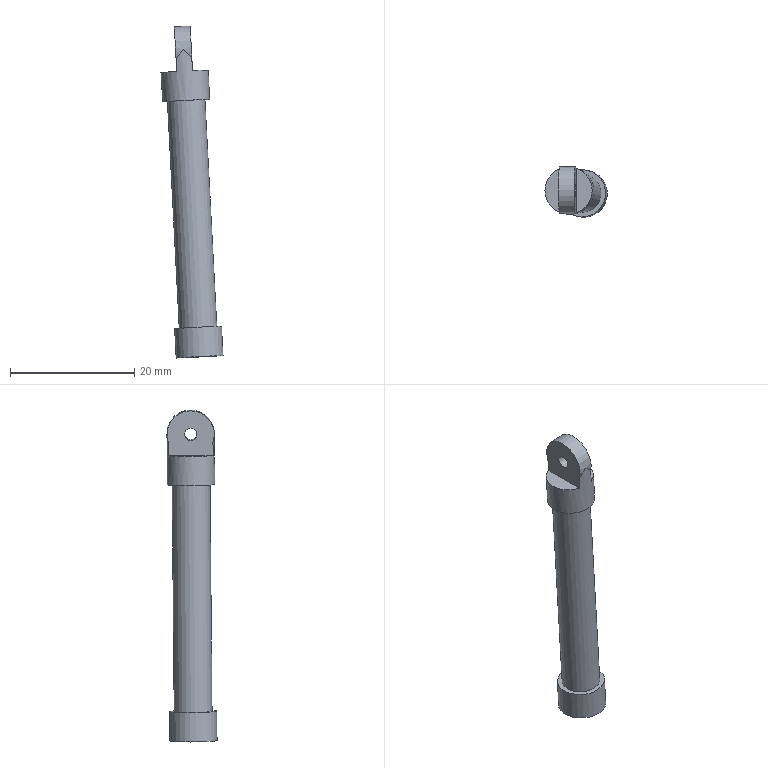Component | NX | CYLINDER_BLOCK | 1 solid | 14 faces | box 10.02 x 8.07 x 53.49 mm | volume 967 mm3 | plane 8 | cylinder 6 | commonest cylinder face diameters 7.62 x3 6.1 x1 2 x1 4.4 x1
STEP:
#1=CARTESIAN_POINT('',(0.,0.,0.));
#2=DIRECTION('',(0.,0.,1.));
#3=DIRECTION('',(1.,0.,0.));
#4=AXIS2_PLACEMENT_3D('',#1,#2,#3);
#5=CARTESIAN_POINT('',(42.989,-37.448,147.365));
#6=VERTEX_POINT('',#5);
#7=CARTESIAN_POINT('',(42.993,-30.264,147.3));
#8=VERTEX_POINT('',#7);
#9=CARTESIAN_POINT('',(44.259,-33.856,147.399));
#10=DIRECTION('',(0.05233,-0.009013,-0.9986));
#11=DIRECTION('',(0.0004717,1.,-0.009));
#12=AXIS2_PLACEMENT_3D('',#9,#10,#11);
#13=CIRCLE('',#12,3.81);
#14=CARTESIAN_POINT('',(44.259,-33.856,147.399));
#15=DIRECTION('',(-0.05233,0.009013,0.9986));
#16=DIRECTION('',(0.0004717,1.,-0.009));
#17=AXIS2_PLACEMENT_3D('',#14,#15,#16);
#18=PLANE('',#17);
#19=CARTESIAN_POINT('',(3.81,0.));
#20=CARTESIAN_POINT('',(3.81,-6.599));
#21=CARTESIAN_POINT('',(-1.905,-3.3));
#22=CARTESIAN_POINT('',(-7.62,-0.));
#23=CARTESIAN_POINT('',(-1.905,3.3));
#24=CARTESIAN_POINT('',(3.81,6.599));
#25=CARTESIAN_POINT('',(3.81,0.));
#26=(BOUNDED_CURVE()B_SPLINE_CURVE(2,(#19,#20,#21,#22,#23,#24,#25),.UNSPECIFIED.,.T.,.F.)B_SPLINE_CURVE_WITH_KNOTS((1,2,2,2,2,1),(-2.094,0.,2.094,4.189,6.283,8.378),.UNSPECIFIED.)CURVE()GEOMETRIC_REPRESENTATION_ITEM()RATIONAL_B_SPLINE_CURVE((1.,0.5,1.,0.5,1.,0.5,1.))REPRESENTATION_ITEM(''));
#27=(GEOMETRIC_REPRESENTATION_CONTEXT(2)PARAMETRIC_REPRESENTATION_CONTEXT()REPRESENTATION_CONTEXT('',''));
#28=DEFINITIONAL_REPRESENTATION('',(#26),#27);
#29=PCURVE('',#18,#28);
#30=CARTESIAN_POINT('',(44.507,-33.899,142.676));
#31=DIRECTION('',(-0.05233,0.009013,0.9986));
#32=DIRECTION('',(0.0004717,1.,-0.009));
#33=AXIS2_PLACEMENT_3D('',#30,#31,#32);
#34=CYLINDRICAL_SURFACE('',#33,3.81);
#35=CARTESIAN_POINT('',(6.283,4.73));
#36=DIRECTION('',(-1.,-0.));
#37=VECTOR('',#36,1.);
#38=LINE('',#35,#37);
#39=(GEOMETRIC_REPRESENTATION_CONTEXT(2)PARAMETRIC_REPRESENTATION_CONTEXT()REPRESENTATION_CONTEXT('',''));
#40=DEFINITIONAL_REPRESENTATION('',(#38),#39);
#41=PCURVE('',#34,#40);
#42=SURFACE_CURVE('',#13,(#29,#41),.PCURVE_S1.);
#43=EDGE_CURVE('',#6,#8,#42,.T.);
#44=ORIENTED_EDGE('',*,*,#43,.F.);
#45=CARTESIAN_POINT('',(42.989,-37.666,147.367));
#46=DIRECTION('',(0.0004717,1.,-0.009));
#47=VECTOR('',#46,1.);
#48=LINE('',#45,#47);
#49=CARTESIAN_POINT('',(-3.81,1.27));
#50=DIRECTION('',(1.,0.));
#51=VECTOR('',#50,1.);
#52=LINE('',#49,#51);
#53=(GEOMETRIC_REPRESENTATION_CONTEXT(2)PARAMETRIC_REPRESENTATION_CONTEXT()REPRESENTATION_CONTEXT('',''));
#54=DEFINITIONAL_REPRESENTATION('',(#52),#53);
#55=PCURVE('',#18,#54);
#56=CARTESIAN_POINT('',(42.989,-37.666,147.367));
#57=DIRECTION('',(0.9986,0.,0.05234));
#58=DIRECTION('',(0.0004717,1.,-0.009));
#59=AXIS2_PLACEMENT_3D('',#56,#57,#58);
#60=PLANE('',#59);
#61=CARTESIAN_POINT('',(0.,0.));
#62=DIRECTION('',(1.,0.));
#63=VECTOR('',#62,1.);
#64=LINE('',#61,#63);
#65=(GEOMETRIC_REPRESENTATION_CONTEXT(2)PARAMETRIC_REPRESENTATION_CONTEXT()REPRESENTATION_CONTEXT('',''));
#66=DEFINITIONAL_REPRESENTATION('',(#64),#65);
#67=PCURVE('',#60,#66);
#68=SURFACE_CURVE('',#48,(#55,#67),.PCURVE_S1.);
#69=EDGE_CURVE('',#6,#8,#68,.T.);
#70=ORIENTED_EDGE('',*,*,#69,.T.);
#71=EDGE_LOOP('',(#44,#70));
#72=FACE_BOUND('',#71,.T.);
#73=ADVANCED_FACE('',(#72),#18,.T.);
#74=CARTESIAN_POINT('',(46.424,-31.179,106.1));
#75=VERTEX_POINT('',#74);
#76=CARTESIAN_POINT('',(46.422,-34.229,106.127));
#77=DIRECTION('',(-0.05233,0.009013,0.9986));
#78=DIRECTION('',(0.0004717,1.,-0.009));
#79=AXIS2_PLACEMENT_3D('',#76,#77,#78);
#80=CIRCLE('',#79,3.05);
#81=CARTESIAN_POINT('',(46.422,-34.229,106.127));
#82=DIRECTION('',(-0.05233,0.009013,0.9986));
#83=DIRECTION('',(0.0004717,1.,-0.009));
#84=AXIS2_PLACEMENT_3D('',#81,#82,#83);
#85=PLANE('',#84);
#86=CARTESIAN_POINT('',(0.,0.));
#87=DIRECTION('',(1.,0.));
#88=AXIS2_PLACEMENT_2D('',#86,#87);
#89=CIRCLE('',#88,3.05);
#90=(GEOMETRIC_REPRESENTATION_CONTEXT(2)PARAMETRIC_REPRESENTATION_CONTEXT()REPRESENTATION_CONTEXT('',''));
#91=DEFINITIONAL_REPRESENTATION('',(#89),#90);
#92=PCURVE('',#85,#91);
#93=CARTESIAN_POINT('',(46.422,-34.229,106.127));
#94=DIRECTION('',(-0.05233,0.009013,0.9986));
#95=DIRECTION('',(0.0004717,1.,-0.009));
#96=AXIS2_PLACEMENT_3D('',#93,#94,#95);
#97=CYLINDRICAL_SURFACE('',#96,3.05);
#98=CARTESIAN_POINT('',(0.,0.));
#99=DIRECTION('',(1.,0.));
#100=VECTOR('',#99,1.);
#101=LINE('',#98,#100);
#102=(GEOMETRIC_REPRESENTATION_CONTEXT(2)PARAMETRIC_REPRESENTATION_CONTEXT()REPRESENTATION_CONTEXT('',''));
#103=DEFINITIONAL_REPRESENTATION('',(#101),#102);
#104=PCURVE('',#97,#103);
#105=SURFACE_CURVE('',#80,(#92,#104),.PCURVE_S1.);
#106=EDGE_CURVE('',#75,#75,#105,.T.);
#107=ORIENTED_EDGE('',*,*,#106,.F.);
#108=EDGE_LOOP('',(#107));
#109=FACE_BOUND('',#108,.T.);
#110=CARTESIAN_POINT('',(46.424,-30.419,106.093));
#111=VERTEX_POINT('',#110);
#112=CARTESIAN_POINT('',(46.422,-34.229,106.127));
#113=DIRECTION('',(0.05233,-0.009013,-0.9986));
#114=DIRECTION('',(0.0004717,1.,-0.009));
#115=AXIS2_PLACEMENT_3D('',#112,#113,#114);
#116=CIRCLE('',#115,3.81);
#117=CARTESIAN_POINT('',(3.81,0.));
#118=CARTESIAN_POINT('',(3.81,-6.599));
#119=CARTESIAN_POINT('',(-1.905,-3.3));
#120=CARTESIAN_POINT('',(-7.62,-0.));
#121=CARTESIAN_POINT('',(-1.905,3.3));
#122=CARTESIAN_POINT('',(3.81,6.599));
#123=CARTESIAN_POINT('',(3.81,0.));
#124=(BOUNDED_CURVE()B_SPLINE_CURVE(2,(#117,#118,#119,#120,#121,#122,#123),.UNSPECIFIED.,.T.,.F.)B_SPLINE_CURVE_WITH_KNOTS((1,2,2,2,2,1),(-2.094,0.,2.094,4.189,6.283,8.378),.UNSPECIFIED.)CURVE()GEOMETRIC_REPRESENTATION_ITEM()RATIONAL_B_SPLINE_CURVE((1.,0.5,1.,0.5,1.,0.5,1.))REPRESENTATION_ITEM(''));
#125=(GEOMETRIC_REPRESENTATION_CONTEXT(2)PARAMETRIC_REPRESENTATION_CONTEXT()REPRESENTATION_CONTEXT('',''));
#126=DEFINITIONAL_REPRESENTATION('',(#124),#125);
#127=PCURVE('',#85,#126);
#128=CARTESIAN_POINT('',(46.67,-34.272,101.404));
#129=DIRECTION('',(-0.05233,0.009013,0.9986));
#130=DIRECTION('',(0.0004717,1.,-0.009));
#131=AXIS2_PLACEMENT_3D('',#128,#129,#130);
#132=CYLINDRICAL_SURFACE('',#131,3.81);
#133=CARTESIAN_POINT('',(6.283,4.73));
#134=DIRECTION('',(-1.,0.));
#135=VECTOR('',#134,1.);
#136=LINE('',#133,#135);
#137=(GEOMETRIC_REPRESENTATION_CONTEXT(2)PARAMETRIC_REPRESENTATION_CONTEXT()REPRESENTATION_CONTEXT('',''));
#138=DEFINITIONAL_REPRESENTATION('',(#136),#137);
#139=PCURVE('',#132,#138);
#140=SURFACE_CURVE('',#116,(#127,#139),.PCURVE_S1.);
#141=EDGE_CURVE('',#111,#111,#140,.T.);
#142=ORIENTED_EDGE('',*,*,#141,.F.);
#143=EDGE_LOOP('',(#142));
#144=FACE_BOUND('',#143,.T.);
#145=ADVANCED_FACE('',(#109,#144),#85,.T.);
#146=CARTESIAN_POINT('',(46.671,-32.072,101.384));
#147=VERTEX_POINT('',#146);
#148=CARTESIAN_POINT('',(46.67,-34.272,101.404));
#149=DIRECTION('',(-0.05233,0.009013,0.9986));
#150=DIRECTION('',(0.0004717,1.,-0.009));
#151=AXIS2_PLACEMENT_3D('',#148,#149,#150);
#152=CIRCLE('',#151,2.2);
#153=CARTESIAN_POINT('',(46.67,-34.272,101.404));
#154=DIRECTION('',(0.05233,-0.009013,-0.9986));
#155=DIRECTION('',(-0.0004717,-1.,0.009));
#156=AXIS2_PLACEMENT_3D('',#153,#154,#155);
#157=PLANE('',#156);
#158=CARTESIAN_POINT('',(-2.2,0.));
#159=CARTESIAN_POINT('',(-2.2,3.811));
#160=CARTESIAN_POINT('',(1.1,1.905));
#161=CARTESIAN_POINT('',(4.4,-0.));
#162=CARTESIAN_POINT('',(1.1,-1.905));
#163=CARTESIAN_POINT('',(-2.2,-3.811));
#164=CARTESIAN_POINT('',(-2.2,0.));
#165=(BOUNDED_CURVE()B_SPLINE_CURVE(2,(#158,#159,#160,#161,#162,#163,#164),.UNSPECIFIED.,.T.,.F.)B_SPLINE_CURVE_WITH_KNOTS((1,2,2,2,2,1),(-2.094,0.,2.094,4.189,6.283,8.378),.UNSPECIFIED.)CURVE()GEOMETRIC_REPRESENTATION_ITEM()RATIONAL_B_SPLINE_CURVE((1.,0.5,1.,0.5,1.,0.5,1.))REPRESENTATION_ITEM(''));
#166=(GEOMETRIC_REPRESENTATION_CONTEXT(2)PARAMETRIC_REPRESENTATION_CONTEXT()REPRESENTATION_CONTEXT('',''));
#167=DEFINITIONAL_REPRESENTATION('',(#165),#166);
#168=PCURVE('',#157,#167);
#169=CARTESIAN_POINT('',(46.67,-34.272,101.404));
#170=DIRECTION('',(-0.05233,0.009013,0.9986));
#171=DIRECTION('',(0.0004717,1.,-0.009));
#172=AXIS2_PLACEMENT_3D('',#169,#170,#171);
#173=CYLINDRICAL_SURFACE('',#172,2.2);
#174=CARTESIAN_POINT('',(0.,0.));
#175=DIRECTION('',(1.,0.));
#176=VECTOR('',#175,1.);
#177=LINE('',#174,#176);
#178=(GEOMETRIC_REPRESENTATION_CONTEXT(2)PARAMETRIC_REPRESENTATION_CONTEXT()REPRESENTATION_CONTEXT('',''));
#179=DEFINITIONAL_REPRESENTATION('',(#177),#178);
#180=PCURVE('',#173,#179);
#181=SURFACE_CURVE('',#152,(#168,#180),.PCURVE_S1.);
#182=EDGE_CURVE('',#147,#147,#181,.T.);
#183=ORIENTED_EDGE('',*,*,#182,.T.);
#184=EDGE_LOOP('',(#183));
#185=FACE_BOUND('',#184,.T.);
#186=CARTESIAN_POINT('',(46.671,-30.462,101.37));
#187=VERTEX_POINT('',#186);
#188=CARTESIAN_POINT('',(46.67,-34.272,101.404));
#189=DIRECTION('',(-0.05233,0.009013,0.9986));
#190=DIRECTION('',(0.0004717,1.,-0.009));
#191=AXIS2_PLACEMENT_3D('',#188,#189,#190);
#192=CIRCLE('',#191,3.81);
#193=CARTESIAN_POINT('',(-3.81,0.));
#194=CARTESIAN_POINT('',(-3.81,6.599));
#195=CARTESIAN_POINT('',(1.905,3.3));
#196=CARTESIAN_POINT('',(7.62,-0.));
#197=CARTESIAN_POINT('',(1.905,-3.3));
#198=CARTESIAN_POINT('',(-3.81,-6.599));
#199=CARTESIAN_POINT('',(-3.81,0.));
#200=(BOUNDED_CURVE()B_SPLINE_CURVE(2,(#193,#194,#195,#196,#197,#198,#199),.UNSPECIFIED.,.T.,.F.)B_SPLINE_CURVE_WITH_KNOTS((1,2,2,2,2,1),(-2.094,0.,2.094,4.189,6.283,8.378),.UNSPECIFIED.)CURVE()GEOMETRIC_REPRESENTATION_ITEM()RATIONAL_B_SPLINE_CURVE((1.,0.5,1.,0.5,1.,0.5,1.))REPRESENTATION_ITEM(''));
#201=(GEOMETRIC_REPRESENTATION_CONTEXT(2)PARAMETRIC_REPRESENTATION_CONTEXT()REPRESENTATION_CONTEXT('',''));
#202=DEFINITIONAL_REPRESENTATION('',(#200),#201);
#203=PCURVE('',#157,#202);
#204=CARTESIAN_POINT('',(0.,0.));
#205=DIRECTION('',(1.,0.));
#206=VECTOR('',#205,1.);
#207=LINE('',#204,#206);
#208=(GEOMETRIC_REPRESENTATION_CONTEXT(2)PARAMETRIC_REPRESENTATION_CONTEXT()REPRESENTATION_CONTEXT('',''));
#209=DEFINITIONAL_REPRESENTATION('',(#207),#208);
#210=PCURVE('',#132,#209);
#211=SURFACE_CURVE('',#192,(#203,#210),.PCURVE_S1.);
#212=EDGE_CURVE('',#187,#187,#211,.T.);
#213=ORIENTED_EDGE('',*,*,#212,.F.);
#214=EDGE_LOOP('',(#213));
#215=FACE_BOUND('',#214,.T.);
#216=ADVANCED_FACE('',(#185,#215),#157,.T.);
#217=ORIENTED_EDGE('',*,*,#141,.T.);
#218=CARTESIAN_POINT('',(46.671,-30.462,101.37));
#219=CARTESIAN_POINT('',(46.424,-30.419,106.093));
#220=B_SPLINE_CURVE_WITH_KNOTS('',1,(#218,#219),.UNSPECIFIED.,.F.,.F.,(2,2),(0.,4.73),.PIECEWISE_BEZIER_KNOTS.);
#221=CARTESIAN_POINT('',(0.,0.));
#222=DIRECTION('',(0.,1.));
#223=VECTOR('',#222,1.);
#224=LINE('',#221,#223);
#225=(GEOMETRIC_REPRESENTATION_CONTEXT(2)PARAMETRIC_REPRESENTATION_CONTEXT()REPRESENTATION_CONTEXT('',''));
#226=DEFINITIONAL_REPRESENTATION('',(#224),#225);
#227=PCURVE('',#132,#226);
#228=CARTESIAN_POINT('',(6.283,0.));
#229=DIRECTION('',(0.,1.));
#230=VECTOR('',#229,1.);
#231=LINE('',#228,#230);
#232=(GEOMETRIC_REPRESENTATION_CONTEXT(2)PARAMETRIC_REPRESENTATION_CONTEXT()REPRESENTATION_CONTEXT('',''));
#233=DEFINITIONAL_REPRESENTATION('',(#231),#232);
#234=PCURVE('',#132,#233);
#235=SEAM_CURVE('',#220,(#227,#234),.PCURVE_S1.);
#236=EDGE_CURVE('',#187,#111,#235,.T.);
#237=ORIENTED_EDGE('',*,*,#236,.F.);
#238=ORIENTED_EDGE('',*,*,#212,.T.);
#239=ORIENTED_EDGE('',*,*,#236,.T.);
#240=EDGE_LOOP('',(#217,#237,#238,#239));
#241=FACE_BOUND('',#240,.T.);
#242=ADVANCED_FACE('',(#241),#132,.T.);
#243=CARTESIAN_POINT('',(44.508,-30.849,142.648));
#244=VERTEX_POINT('',#243);
#245=CARTESIAN_POINT('',(44.505,-36.949,142.703));
#246=VERTEX_POINT('',#245);
#247=CARTESIAN_POINT('',(44.507,-33.899,142.676));
#248=DIRECTION('',(-0.05233,0.009013,0.9986));
#249=DIRECTION('',(-0.0004717,-1.,0.009));
#250=AXIS2_PLACEMENT_3D('',#247,#248,#249);
#251=CIRCLE('',#250,3.05);
#252=CARTESIAN_POINT('',(-3.142,36.6));
#253=DIRECTION('',(1.,0.));
#254=VECTOR('',#253,1.);
#255=LINE('',#252,#254);
#256=(GEOMETRIC_REPRESENTATION_CONTEXT(2)PARAMETRIC_REPRESENTATION_CONTEXT()REPRESENTATION_CONTEXT('',''));
#257=DEFINITIONAL_REPRESENTATION('',(#255),#256);
#258=PCURVE('',#97,#257);
#259=CARTESIAN_POINT('',(44.507,-33.899,142.676));
#260=DIRECTION('',(0.05233,-0.009013,-0.9986));
#261=DIRECTION('',(-0.0004717,-1.,0.009));
#262=AXIS2_PLACEMENT_3D('',#259,#260,#261);
#263=PLANE('',#262);
#264=CARTESIAN_POINT('',(3.05,-0.));
#265=CARTESIAN_POINT('',(3.05,-5.283));
#266=CARTESIAN_POINT('',(-1.525,-2.641));
#267=CARTESIAN_POINT('',(-6.1,0.));
#268=CARTESIAN_POINT('',(-1.525,2.641));
#269=CARTESIAN_POINT('',(3.05,5.283));
#270=CARTESIAN_POINT('',(3.05,-0.));
#271=(BOUNDED_CURVE()B_SPLINE_CURVE(2,(#264,#265,#266,#267,#268,#269,#270),.UNSPECIFIED.,.T.,.F.)B_SPLINE_CURVE_WITH_KNOTS((1,2,2,2,2,1),(-2.094,0.,2.094,4.189,6.283,8.378),.UNSPECIFIED.)CURVE()GEOMETRIC_REPRESENTATION_ITEM()RATIONAL_B_SPLINE_CURVE((1.,0.5,1.,0.5,1.,0.5,1.))REPRESENTATION_ITEM(''));
#272=(GEOMETRIC_REPRESENTATION_CONTEXT(2)PARAMETRIC_REPRESENTATION_CONTEXT()REPRESENTATION_CONTEXT('',''));
#273=DEFINITIONAL_REPRESENTATION('',(#271),#272);
#274=PCURVE('',#263,#273);
#275=SURFACE_CURVE('',#251,(#258,#274),.PCURVE_S1.);
#276=EDGE_CURVE('',#244,#246,#275,.T.);
#277=ORIENTED_EDGE('',*,*,#276,.F.);
#278=CARTESIAN_POINT('',(46.424,-31.179,106.1));
#279=CARTESIAN_POINT('',(44.508,-30.849,142.648));
#280=B_SPLINE_CURVE_WITH_KNOTS('',1,(#278,#279),.UNSPECIFIED.,.F.,.F.,(2,2),(0.,36.6),.PIECEWISE_BEZIER_KNOTS.);
#281=CARTESIAN_POINT('',(0.,0.));
#282=DIRECTION('',(0.,1.));
#283=VECTOR('',#282,1.);
#284=LINE('',#281,#283);
#285=(GEOMETRIC_REPRESENTATION_CONTEXT(2)PARAMETRIC_REPRESENTATION_CONTEXT()REPRESENTATION_CONTEXT('',''));
#286=DEFINITIONAL_REPRESENTATION('',(#284),#285);
#287=PCURVE('',#97,#286);
#288=CARTESIAN_POINT('',(6.283,0.));
#289=DIRECTION('',(0.,1.));
#290=VECTOR('',#289,1.);
#291=LINE('',#288,#290);
#292=(GEOMETRIC_REPRESENTATION_CONTEXT(2)PARAMETRIC_REPRESENTATION_CONTEXT()REPRESENTATION_CONTEXT('',''));
#293=DEFINITIONAL_REPRESENTATION('',(#291),#292);
#294=PCURVE('',#97,#293);
#295=SEAM_CURVE('',#280,(#287,#294),.PCURVE_S1.);
#296=EDGE_CURVE('',#75,#244,#295,.T.);
#297=ORIENTED_EDGE('',*,*,#296,.F.);
#298=ORIENTED_EDGE('',*,*,#106,.T.);
#299=ORIENTED_EDGE('',*,*,#296,.T.);
#300=CARTESIAN_POINT('',(44.507,-33.899,142.676));
#301=DIRECTION('',(-0.05233,0.009013,0.9986));
#302=DIRECTION('',(-0.0004717,-1.,0.009));
#303=AXIS2_PLACEMENT_3D('',#300,#301,#302);
#304=CIRCLE('',#303,3.05);
#305=CARTESIAN_POINT('',(3.142,36.6));
#306=DIRECTION('',(1.,0.));
#307=VECTOR('',#306,1.);
#308=LINE('',#305,#307);
#309=(GEOMETRIC_REPRESENTATION_CONTEXT(2)PARAMETRIC_REPRESENTATION_CONTEXT()REPRESENTATION_CONTEXT('',''));
#310=DEFINITIONAL_REPRESENTATION('',(#308),#309);
#311=PCURVE('',#97,#310);
#312=CARTESIAN_POINT('',(3.05,-0.));
#313=CARTESIAN_POINT('',(3.05,-5.283));
#314=CARTESIAN_POINT('',(-1.525,-2.641));
#315=CARTESIAN_POINT('',(-6.1,0.));
#316=CARTESIAN_POINT('',(-1.525,2.641));
#317=CARTESIAN_POINT('',(3.05,5.283));
#318=CARTESIAN_POINT('',(3.05,-0.));
#319=(BOUNDED_CURVE()B_SPLINE_CURVE(2,(#312,#313,#314,#315,#316,#317,#318),.UNSPECIFIED.,.T.,.F.)B_SPLINE_CURVE_WITH_KNOTS((1,2,2,2,2,1),(-2.094,0.,2.094,4.189,6.283,8.378),.UNSPECIFIED.)CURVE()GEOMETRIC_REPRESENTATION_ITEM()RATIONAL_B_SPLINE_CURVE((1.,0.5,1.,0.5,1.,0.5,1.))REPRESENTATION_ITEM(''));
#320=(GEOMETRIC_REPRESENTATION_CONTEXT(2)PARAMETRIC_REPRESENTATION_CONTEXT()REPRESENTATION_CONTEXT('',''));
#321=DEFINITIONAL_REPRESENTATION('',(#319),#320);
#322=PCURVE('',#263,#321);
#323=SURFACE_CURVE('',#304,(#311,#322),.PCURVE_S1.);
#324=EDGE_CURVE('',#246,#244,#323,.T.);
#325=ORIENTED_EDGE('',*,*,#324,.F.);
#326=EDGE_LOOP('',(#277,#297,#298,#299,#325));
#327=FACE_BOUND('',#326,.T.);
#328=ADVANCED_FACE('',(#327),#97,.T.);
#329=CARTESIAN_POINT('',(45.526,-37.448,147.498));
#330=VERTEX_POINT('',#329);
#331=CARTESIAN_POINT('',(45.529,-30.264,147.433));
#332=VERTEX_POINT('',#331);
#333=CARTESIAN_POINT('',(45.526,-37.666,147.5));
#334=DIRECTION('',(0.0004717,1.,-0.009));
#335=VECTOR('',#334,1.);
#336=LINE('',#333,#335);
#337=CARTESIAN_POINT('',(44.259,-33.856,147.399));
#338=DIRECTION('',(-0.05233,0.009013,0.9986));
#339=DIRECTION('',(0.0004717,1.,-0.009));
#340=AXIS2_PLACEMENT_3D('',#337,#338,#339);
#341=PLANE('',#340);
#342=CARTESIAN_POINT('',(-3.81,-1.27));
#343=DIRECTION('',(1.,0.));
#344=VECTOR('',#343,1.);
#345=LINE('',#342,#344);
#346=(GEOMETRIC_REPRESENTATION_CONTEXT(2)PARAMETRIC_REPRESENTATION_CONTEXT()REPRESENTATION_CONTEXT('',''));
#347=DEFINITIONAL_REPRESENTATION('',(#345),#346);
#348=PCURVE('',#341,#347);
#349=CARTESIAN_POINT('',(45.526,-37.666,147.5));
#350=DIRECTION('',(0.9986,0.,0.05234));
#351=DIRECTION('',(0.0004717,1.,-0.009));
#352=AXIS2_PLACEMENT_3D('',#349,#350,#351);
#353=PLANE('',#352);
#354=CARTESIAN_POINT('',(0.,0.));
#355=DIRECTION('',(1.,0.));
#356=VECTOR('',#355,1.);
#357=LINE('',#354,#356);
#358=(GEOMETRIC_REPRESENTATION_CONTEXT(2)PARAMETRIC_REPRESENTATION_CONTEXT()REPRESENTATION_CONTEXT('',''));
#359=DEFINITIONAL_REPRESENTATION('',(#357),#358);
#360=PCURVE('',#353,#359);
#361=SURFACE_CURVE('',#336,(#348,#360),.PCURVE_S1.);
#362=EDGE_CURVE('',#330,#332,#361,.T.);
#363=ORIENTED_EDGE('',*,*,#362,.F.);
#364=CARTESIAN_POINT('',(44.259,-33.856,147.399));
#365=DIRECTION('',(0.05233,-0.009013,-0.9986));
#366=DIRECTION('',(0.0004717,1.,-0.009));
#367=AXIS2_PLACEMENT_3D('',#364,#365,#366);
#368=CIRCLE('',#367,3.81);
#369=CARTESIAN_POINT('',(3.81,0.));
#370=CARTESIAN_POINT('',(3.81,-6.599));
#371=CARTESIAN_POINT('',(-1.905,-3.3));
#372=CARTESIAN_POINT('',(-7.62,-0.));
#373=CARTESIAN_POINT('',(-1.905,3.3));
#374=CARTESIAN_POINT('',(3.81,6.599));
#375=CARTESIAN_POINT('',(3.81,0.));
#376=(BOUNDED_CURVE()B_SPLINE_CURVE(2,(#369,#370,#371,#372,#373,#374,#375),.UNSPECIFIED.,.T.,.F.)B_SPLINE_CURVE_WITH_KNOTS((1,2,2,2,2,1),(-2.094,0.,2.094,4.189,6.283,8.378),.UNSPECIFIED.)CURVE()GEOMETRIC_REPRESENTATION_ITEM()RATIONAL_B_SPLINE_CURVE((1.,0.5,1.,0.5,1.,0.5,1.))REPRESENTATION_ITEM(''));
#377=(GEOMETRIC_REPRESENTATION_CONTEXT(2)PARAMETRIC_REPRESENTATION_CONTEXT()REPRESENTATION_CONTEXT('',''));
#378=DEFINITIONAL_REPRESENTATION('',(#376),#377);
#379=PCURVE('',#341,#378);
#380=CARTESIAN_POINT('',(6.283,4.73));
#381=DIRECTION('',(-1.,0.));
#382=VECTOR('',#381,1.);
#383=LINE('',#380,#382);
#384=(GEOMETRIC_REPRESENTATION_CONTEXT(2)PARAMETRIC_REPRESENTATION_CONTEXT()REPRESENTATION_CONTEXT('',''));
#385=DEFINITIONAL_REPRESENTATION('',(#383),#384);
#386=PCURVE('',#34,#385);
#387=SURFACE_CURVE('',#368,(#379,#386),.PCURVE_S1.);
#388=EDGE_CURVE('',#332,#330,#387,.T.);
#389=ORIENTED_EDGE('',*,*,#388,.F.);
#390=EDGE_LOOP('',(#363,#389));
#391=FACE_BOUND('',#390,.T.);
#392=ADVANCED_FACE('',(#391),#341,.T.);
#393=ORIENTED_EDGE('',*,*,#324,.T.);
#394=ORIENTED_EDGE('',*,*,#276,.T.);
#395=EDGE_LOOP('',(#393,#394));
#396=FACE_BOUND('',#395,.T.);
#397=CARTESIAN_POINT('',(44.509,-30.089,142.642));
#398=VERTEX_POINT('',#397);
#399=CARTESIAN_POINT('',(44.507,-33.899,142.676));
#400=DIRECTION('',(-0.05233,0.009013,0.9986));
#401=DIRECTION('',(0.0004717,1.,-0.009));
#402=AXIS2_PLACEMENT_3D('',#399,#400,#401);
#403=CIRCLE('',#402,3.81);
#404=CARTESIAN_POINT('',(-3.81,0.));
#405=CARTESIAN_POINT('',(-3.81,6.599));
#406=CARTESIAN_POINT('',(1.905,3.3));
#407=CARTESIAN_POINT('',(7.62,-0.));
#408=CARTESIAN_POINT('',(1.905,-3.3));
#409=CARTESIAN_POINT('',(-3.81,-6.599));
#410=CARTESIAN_POINT('',(-3.81,0.));
#411=(BOUNDED_CURVE()B_SPLINE_CURVE(2,(#404,#405,#406,#407,#408,#409,#410),.UNSPECIFIED.,.T.,.F.)B_SPLINE_CURVE_WITH_KNOTS((1,2,2,2,2,1),(-2.094,0.,2.094,4.189,6.283,8.378),.UNSPECIFIED.)CURVE()GEOMETRIC_REPRESENTATION_ITEM()RATIONAL_B_SPLINE_CURVE((1.,0.5,1.,0.5,1.,0.5,1.))REPRESENTATION_ITEM(''));
#412=(GEOMETRIC_REPRESENTATION_CONTEXT(2)PARAMETRIC_REPRESENTATION_CONTEXT()REPRESENTATION_CONTEXT('',''));
#413=DEFINITIONAL_REPRESENTATION('',(#411),#412);
#414=PCURVE('',#263,#413);
#415=CARTESIAN_POINT('',(0.,0.));
#416=DIRECTION('',(1.,0.));
#417=VECTOR('',#416,1.);
#418=LINE('',#415,#417);
#419=(GEOMETRIC_REPRESENTATION_CONTEXT(2)PARAMETRIC_REPRESENTATION_CONTEXT()REPRESENTATION_CONTEXT('',''));
#420=DEFINITIONAL_REPRESENTATION('',(#418),#419);
#421=PCURVE('',#34,#420);
#422=SURFACE_CURVE('',#403,(#414,#421),.PCURVE_S1.);
#423=EDGE_CURVE('',#398,#398,#422,.T.);
#424=ORIENTED_EDGE('',*,*,#423,.F.);
#425=EDGE_LOOP('',(#424));
#426=FACE_BOUND('',#425,.T.);
#427=ADVANCED_FACE('',(#396,#426),#263,.T.);
#428=CARTESIAN_POINT('',(42.876,-37.429,149.522));
#429=VERTEX_POINT('',#428);
#430=CARTESIAN_POINT('',(44.078,-37.635,150.859));
#431=VERTEX_POINT('',#430);
#432=CARTESIAN_POINT('',(44.08,-33.825,150.824));
#433=DIRECTION('',(-0.7431,0.006373,0.6691));
#434=DIRECTION('',(0.6691,0.006373,0.7431));
#435=AXIS2_PLACEMENT_3D('',#432,#433,#434);
#436=ELLIPSE('',#435,5.388,3.81);
#437=CARTESIAN_POINT('',(2.802,6.89));
#438=CARTESIAN_POINT('',(3.142,8.16));
#439=B_SPLINE_CURVE_WITH_KNOTS('',1,(#437,#438),.UNSPECIFIED.,.F.,.F.,(2,2),(4.373,4.712),.PIECEWISE_BEZIER_KNOTS.);
#440=(GEOMETRIC_REPRESENTATION_CONTEXT(2)PARAMETRIC_REPRESENTATION_CONTEXT()REPRESENTATION_CONTEXT('',''));
#441=DEFINITIONAL_REPRESENTATION('',(#439),#440);
#442=PCURVE('',#34,#441);
#443=CARTESIAN_POINT('',(45.348,-33.825,150.891));
#444=DIRECTION('',(-0.9986,-0.,-0.05234));
#445=DIRECTION('',(0.0004717,1.,-0.009));
#446=AXIS2_PLACEMENT_3D('',#443,#444,#445);
#447=CYLINDRICAL_SURFACE('',#446,3.81);
#448=CARTESIAN_POINT('',(2.802,2.54));
#449=CARTESIAN_POINT('',(3.142,1.27));
#450=B_SPLINE_CURVE_WITH_KNOTS('',1,(#448,#449),.UNSPECIFIED.,.F.,.F.,(2,2),(4.373,4.712),.PIECEWISE_BEZIER_KNOTS.);
#451=(GEOMETRIC_REPRESENTATION_CONTEXT(2)PARAMETRIC_REPRESENTATION_CONTEXT()REPRESENTATION_CONTEXT('',''));
#452=DEFINITIONAL_REPRESENTATION('',(#450),#451);
#453=PCURVE('',#447,#452);
#454=SURFACE_CURVE('',#436,(#442,#453),.PCURVE_S1.);
#455=EDGE_CURVE('',#429,#431,#454,.T.);
#456=ORIENTED_EDGE('',*,*,#455,.F.);
#457=CARTESIAN_POINT('',(42.899,-37.433,149.078));
#458=DIRECTION('',(0.05233,-0.009013,-0.9986));
#459=VECTOR('',#458,1.);
#460=LINE('',#457,#459);
#461=CARTESIAN_POINT('',(2.802,6.445));
#462=DIRECTION('',(0.,-1.));
#463=VECTOR('',#462,1.);
#464=LINE('',#461,#463);
#465=(GEOMETRIC_REPRESENTATION_CONTEXT(2)PARAMETRIC_REPRESENTATION_CONTEXT()REPRESENTATION_CONTEXT('',''));
#466=DEFINITIONAL_REPRESENTATION('',(#464),#465);
#467=PCURVE('',#34,#466);
#468=CARTESIAN_POINT('',(0.2179,1.715));
#469=DIRECTION('',(0.,-1.));
#470=VECTOR('',#469,1.);
#471=LINE('',#468,#470);
#472=(GEOMETRIC_REPRESENTATION_CONTEXT(2)PARAMETRIC_REPRESENTATION_CONTEXT()REPRESENTATION_CONTEXT('',''));
#473=DEFINITIONAL_REPRESENTATION('',(#471),#472);
#474=PCURVE('',#60,#473);
#475=SURFACE_CURVE('',#460,(#467,#474),.PCURVE_S1.);
#476=EDGE_CURVE('',#429,#6,#475,.T.);
#477=ORIENTED_EDGE('',*,*,#476,.T.);
#478=ORIENTED_EDGE('',*,*,#43,.T.);
#479=CARTESIAN_POINT('',(42.88,-30.245,149.457));
#480=VERTEX_POINT('',#479);
#481=CARTESIAN_POINT('',(42.903,-30.249,149.013));
#482=DIRECTION('',(-0.05233,0.009013,0.9986));
#483=VECTOR('',#482,1.);
#484=LINE('',#481,#483);
#485=CARTESIAN_POINT('',(0.3398,6.445));
#486=DIRECTION('',(0.,1.));
#487=VECTOR('',#486,1.);
#488=LINE('',#485,#487);
#489=(GEOMETRIC_REPRESENTATION_CONTEXT(2)PARAMETRIC_REPRESENTATION_CONTEXT()REPRESENTATION_CONTEXT('',''));
#490=DEFINITIONAL_REPRESENTATION('',(#488),#489);
#491=PCURVE('',#34,#490);
#492=CARTESIAN_POINT('',(7.402,1.715));
#493=DIRECTION('',(-0.,1.));
#494=VECTOR('',#493,1.);
#495=LINE('',#492,#494);
#496=(GEOMETRIC_REPRESENTATION_CONTEXT(2)PARAMETRIC_REPRESENTATION_CONTEXT()REPRESENTATION_CONTEXT('',''));
#497=DEFINITIONAL_REPRESENTATION('',(#495),#496);
#498=PCURVE('',#60,#497);
#499=SURFACE_CURVE('',#484,(#491,#498),.PCURVE_S1.);
#500=EDGE_CURVE('',#8,#480,#499,.T.);
#501=ORIENTED_EDGE('',*,*,#500,.T.);
#502=CARTESIAN_POINT('',(44.081,-30.016,150.79));
#503=VERTEX_POINT('',#502);
#504=CARTESIAN_POINT('',(44.08,-33.825,150.824));
#505=DIRECTION('',(-0.7431,0.006373,0.6691));
#506=DIRECTION('',(0.6691,0.006373,0.7431));
#507=AXIS2_PLACEMENT_3D('',#504,#505,#506);
#508=ELLIPSE('',#507,5.388,3.81);
#509=CARTESIAN_POINT('',(0.,8.16));
#510=CARTESIAN_POINT('',(0.3398,6.89));
#511=B_SPLINE_CURVE_WITH_KNOTS('',1,(#509,#510),.UNSPECIFIED.,.F.,.F.,(2,2),(1.571,1.911),.PIECEWISE_BEZIER_KNOTS.);
#512=(GEOMETRIC_REPRESENTATION_CONTEXT(2)PARAMETRIC_REPRESENTATION_CONTEXT()REPRESENTATION_CONTEXT('',''));
#513=DEFINITIONAL_REPRESENTATION('',(#511),#512);
#514=PCURVE('',#34,#513);
#515=CARTESIAN_POINT('',(6.283,1.27));
#516=CARTESIAN_POINT('',(6.623,2.54));
#517=B_SPLINE_CURVE_WITH_KNOTS('',1,(#515,#516),.UNSPECIFIED.,.F.,.F.,(2,2),(1.571,1.911),.PIECEWISE_BEZIER_KNOTS.);
#518=(GEOMETRIC_REPRESENTATION_CONTEXT(2)PARAMETRIC_REPRESENTATION_CONTEXT()REPRESENTATION_CONTEXT('',''));
#519=DEFINITIONAL_REPRESENTATION('',(#517),#518);
#520=PCURVE('',#447,#519);
#521=SURFACE_CURVE('',#508,(#514,#520),.PCURVE_S1.);
#522=EDGE_CURVE('',#503,#480,#521,.T.);
#523=ORIENTED_EDGE('',*,*,#522,.F.);
#524=CARTESIAN_POINT('',(44.509,-30.089,142.642));
#525=CARTESIAN_POINT('',(44.081,-30.016,150.79));
#526=B_SPLINE_CURVE_WITH_KNOTS('',1,(#524,#525),.UNSPECIFIED.,.F.,.F.,(2,2),(0.,8.16),.PIECEWISE_BEZIER_KNOTS.);
#527=CARTESIAN_POINT('',(0.,0.));
#528=DIRECTION('',(0.,1.));
#529=VECTOR('',#528,1.);
#530=LINE('',#527,#529);
#531=(GEOMETRIC_REPRESENTATION_CONTEXT(2)PARAMETRIC_REPRESENTATION_CONTEXT()REPRESENTATION_CONTEXT('',''));
#532=DEFINITIONAL_REPRESENTATION('',(#530),#531);
#533=PCURVE('',#34,#532);
#534=CARTESIAN_POINT('',(6.283,0.));
#535=DIRECTION('',(0.,1.));
#536=VECTOR('',#535,1.);
#537=LINE('',#534,#536);
#538=(GEOMETRIC_REPRESENTATION_CONTEXT(2)PARAMETRIC_REPRESENTATION_CONTEXT()REPRESENTATION_CONTEXT('',''));
#539=DEFINITIONAL_REPRESENTATION('',(#537),#538);
#540=PCURVE('',#34,#539);
#541=SEAM_CURVE('',#526,(#533,#540),.PCURVE_S1.);
#542=EDGE_CURVE('',#398,#503,#541,.T.);
#543=ORIENTED_EDGE('',*,*,#542,.F.);
#544=ORIENTED_EDGE('',*,*,#423,.T.);
#545=ORIENTED_EDGE('',*,*,#542,.T.);
#546=CARTESIAN_POINT('',(45.416,-30.245,149.59));
#547=VERTEX_POINT('',#546);
#548=CARTESIAN_POINT('',(44.08,-33.825,150.824));
#549=DIRECTION('',(0.6691,0.006373,0.7431));
#550=DIRECTION('',(-0.7431,0.006373,0.6691));
#551=AXIS2_PLACEMENT_3D('',#548,#549,#550);
#552=ELLIPSE('',#551,5.388,3.81);
#553=CARTESIAN_POINT('',(5.943,6.89));
#554=CARTESIAN_POINT('',(6.283,8.16));
#555=B_SPLINE_CURVE_WITH_KNOTS('',1,(#553,#554),.UNSPECIFIED.,.F.,.F.,(2,2),(4.373,4.712),.PIECEWISE_BEZIER_KNOTS.);
#556=(GEOMETRIC_REPRESENTATION_CONTEXT(2)PARAMETRIC_REPRESENTATION_CONTEXT()REPRESENTATION_CONTEXT('',''));
#557=DEFINITIONAL_REPRESENTATION('',(#555),#556);
#558=PCURVE('',#34,#557);
#559=CARTESIAN_POINT('',(6.623,0.));
#560=CARTESIAN_POINT('',(6.283,1.27));
#561=B_SPLINE_CURVE_WITH_KNOTS('',1,(#559,#560),.UNSPECIFIED.,.F.,.F.,(2,2),(4.373,4.712),.PIECEWISE_BEZIER_KNOTS.);
#562=(GEOMETRIC_REPRESENTATION_CONTEXT(2)PARAMETRIC_REPRESENTATION_CONTEXT()REPRESENTATION_CONTEXT('',''));
#563=DEFINITIONAL_REPRESENTATION('',(#561),#562);
#564=PCURVE('',#447,#563);
#565=SURFACE_CURVE('',#552,(#558,#564),.PCURVE_S1.);
#566=EDGE_CURVE('',#547,#503,#565,.T.);
#567=ORIENTED_EDGE('',*,*,#566,.F.);
#568=CARTESIAN_POINT('',(45.439,-30.249,149.146));
#569=DIRECTION('',(-0.05233,0.009013,0.9986));
#570=VECTOR('',#569,1.);
#571=LINE('',#568,#570);
#572=CARTESIAN_POINT('',(5.943,6.445));
#573=DIRECTION('',(-0.,1.));
#574=VECTOR('',#573,1.);
#575=LINE('',#572,#574);
#576=(GEOMETRIC_REPRESENTATION_CONTEXT(2)PARAMETRIC_REPRESENTATION_CONTEXT()REPRESENTATION_CONTEXT('',''));
#577=DEFINITIONAL_REPRESENTATION('',(#575),#576);
#578=PCURVE('',#34,#577);
#579=CARTESIAN_POINT('',(7.402,1.715));
#580=DIRECTION('',(-0.,1.));
#581=VECTOR('',#580,1.);
#582=LINE('',#579,#581);
#583=(GEOMETRIC_REPRESENTATION_CONTEXT(2)PARAMETRIC_REPRESENTATION_CONTEXT()REPRESENTATION_CONTEXT('',''));
#584=DEFINITIONAL_REPRESENTATION('',(#582),#583);
#585=PCURVE('',#353,#584);
#586=SURFACE_CURVE('',#571,(#578,#585),.PCURVE_S1.);
#587=EDGE_CURVE('',#332,#547,#586,.T.);
#588=ORIENTED_EDGE('',*,*,#587,.F.);
#589=ORIENTED_EDGE('',*,*,#388,.T.);
#590=CARTESIAN_POINT('',(45.413,-37.429,149.655));
#591=VERTEX_POINT('',#590);
#592=CARTESIAN_POINT('',(45.436,-37.433,149.211));
#593=DIRECTION('',(0.05233,-0.009013,-0.9986));
#594=VECTOR('',#593,1.);
#595=LINE('',#592,#594);
#596=CARTESIAN_POINT('',(3.481,6.445));
#597=DIRECTION('',(0.,-1.));
#598=VECTOR('',#597,1.);
#599=LINE('',#596,#598);
#600=(GEOMETRIC_REPRESENTATION_CONTEXT(2)PARAMETRIC_REPRESENTATION_CONTEXT()REPRESENTATION_CONTEXT('',''));
#601=DEFINITIONAL_REPRESENTATION('',(#599),#600);
#602=PCURVE('',#34,#601);
#603=CARTESIAN_POINT('',(0.2179,1.715));
#604=DIRECTION('',(0.,-1.));
#605=VECTOR('',#604,1.);
#606=LINE('',#603,#605);
#607=(GEOMETRIC_REPRESENTATION_CONTEXT(2)PARAMETRIC_REPRESENTATION_CONTEXT()REPRESENTATION_CONTEXT('',''));
#608=DEFINITIONAL_REPRESENTATION('',(#606),#607);
#609=PCURVE('',#353,#608);
#610=SURFACE_CURVE('',#595,(#602,#609),.PCURVE_S1.);
#611=EDGE_CURVE('',#591,#330,#610,.T.);
#612=ORIENTED_EDGE('',*,*,#611,.F.);
#613=CARTESIAN_POINT('',(44.08,-33.825,150.824));
#614=DIRECTION('',(0.6691,0.006373,0.7431));
#615=DIRECTION('',(-0.7431,0.006373,0.6691));
#616=AXIS2_PLACEMENT_3D('',#613,#614,#615);
#617=ELLIPSE('',#616,5.388,3.81);
#618=CARTESIAN_POINT('',(3.142,8.16));
#619=CARTESIAN_POINT('',(3.481,6.89));
#620=B_SPLINE_CURVE_WITH_KNOTS('',1,(#618,#619),.UNSPECIFIED.,.F.,.F.,(2,2),(1.571,1.911),.PIECEWISE_BEZIER_KNOTS.);
#621=(GEOMETRIC_REPRESENTATION_CONTEXT(2)PARAMETRIC_REPRESENTATION_CONTEXT()REPRESENTATION_CONTEXT('',''));
#622=DEFINITIONAL_REPRESENTATION('',(#620),#621);
#623=PCURVE('',#34,#622);
#624=CARTESIAN_POINT('',(3.142,1.27));
#625=CARTESIAN_POINT('',(2.802,0.));
#626=B_SPLINE_CURVE_WITH_KNOTS('',1,(#624,#625),.UNSPECIFIED.,.F.,.F.,(2,2),(1.571,1.911),.PIECEWISE_BEZIER_KNOTS.);
#627=(GEOMETRIC_REPRESENTATION_CONTEXT(2)PARAMETRIC_REPRESENTATION_CONTEXT()REPRESENTATION_CONTEXT('',''));
#628=DEFINITIONAL_REPRESENTATION('',(#626),#627);
#629=PCURVE('',#447,#628);
#630=SURFACE_CURVE('',#617,(#623,#629),.PCURVE_S1.);
#631=EDGE_CURVE('',#431,#591,#630,.T.);
#632=ORIENTED_EDGE('',*,*,#631,.F.);
#633=EDGE_LOOP('',(#456,#477,#478,#501,#523,#543,#544,#545,#567,#588,#589,#612,#632));
#634=FACE_BOUND('',#633,.T.);
#635=ADVANCED_FACE('',(#634),#34,.T.);
#636=CARTESIAN_POINT('',(45.347,-34.825,150.9));
#637=VERTEX_POINT('',#636);
#638=CARTESIAN_POINT('',(45.348,-33.825,150.891));
#639=DIRECTION('',(-0.9986,-0.,-0.05234));
#640=DIRECTION('',(-0.0004717,-1.,0.009));
#641=AXIS2_PLACEMENT_3D('',#638,#639,#640);
#642=CIRCLE('',#641,1.);
#643=CARTESIAN_POINT('',(2.81,3.43));
#644=CARTESIAN_POINT('',(2.81,5.162));
#645=CARTESIAN_POINT('',(4.31,4.296));
#646=CARTESIAN_POINT('',(5.81,3.43));
#647=CARTESIAN_POINT('',(4.31,2.564));
#648=CARTESIAN_POINT('',(2.81,1.698));
#649=CARTESIAN_POINT('',(2.81,3.43));
#650=(BOUNDED_CURVE()B_SPLINE_CURVE(2,(#643,#644,#645,#646,#647,#648,#649),.UNSPECIFIED.,.T.,.F.)B_SPLINE_CURVE_WITH_KNOTS((1,2,2,2,2,1),(-2.094,0.,2.094,4.189,6.283,8.378),.UNSPECIFIED.)CURVE()GEOMETRIC_REPRESENTATION_ITEM()RATIONAL_B_SPLINE_CURVE((1.,0.5,1.,0.5,1.,0.5,1.))REPRESENTATION_ITEM(''));
#651=(GEOMETRIC_REPRESENTATION_CONTEXT(2)PARAMETRIC_REPRESENTATION_CONTEXT()REPRESENTATION_CONTEXT('',''));
#652=DEFINITIONAL_REPRESENTATION('',(#650),#651);
#653=PCURVE('',#353,#652);
#654=CARTESIAN_POINT('',(45.348,-33.825,150.891));
#655=DIRECTION('',(-0.9986,-0.,-0.05234));
#656=DIRECTION('',(-0.0004717,-1.,0.009));
#657=AXIS2_PLACEMENT_3D('',#654,#655,#656);
#658=CYLINDRICAL_SURFACE('',#657,1.);
#659=CARTESIAN_POINT('',(0.,0.));
#660=DIRECTION('',(1.,0.));
#661=VECTOR('',#660,1.);
#662=LINE('',#659,#661);
#663=(GEOMETRIC_REPRESENTATION_CONTEXT(2)PARAMETRIC_REPRESENTATION_CONTEXT()REPRESENTATION_CONTEXT('',''));
#664=DEFINITIONAL_REPRESENTATION('',(#662),#663);
#665=PCURVE('',#658,#664);
#666=SURFACE_CURVE('',#642,(#653,#665),.PCURVE_S1.);
#667=EDGE_CURVE('',#637,#637,#666,.T.);
#668=ORIENTED_EDGE('',*,*,#667,.T.);
#669=EDGE_LOOP('',(#668));
#670=FACE_BOUND('',#669,.T.);
#671=CARTESIAN_POINT('',(45.348,-33.825,150.891));
#672=DIRECTION('',(-0.9986,-0.,-0.05234));
#673=DIRECTION('',(0.0004717,1.,-0.009));
#674=AXIS2_PLACEMENT_3D('',#671,#672,#673);
#675=CIRCLE('',#674,3.81);
#676=CARTESIAN_POINT('',(7.62,3.43));
#677=CARTESIAN_POINT('',(7.62,-3.169));
#678=CARTESIAN_POINT('',(1.905,0.1304));
#679=CARTESIAN_POINT('',(-3.81,3.43));
#680=CARTESIAN_POINT('',(1.905,6.73));
#681=CARTESIAN_POINT('',(7.62,10.029));
#682=CARTESIAN_POINT('',(7.62,3.43));
#683=(BOUNDED_CURVE()B_SPLINE_CURVE(2,(#676,#677,#678,#679,#680,#681,#682),.UNSPECIFIED.,.T.,.F.)B_SPLINE_CURVE_WITH_KNOTS((1,2,2,2,2,1),(-2.094,0.,2.094,4.189,6.283,8.378),.UNSPECIFIED.)CURVE()GEOMETRIC_REPRESENTATION_ITEM()RATIONAL_B_SPLINE_CURVE((1.,0.5,1.,0.5,1.,0.5,1.))REPRESENTATION_ITEM(''));
#684=(GEOMETRIC_REPRESENTATION_CONTEXT(2)PARAMETRIC_REPRESENTATION_CONTEXT()REPRESENTATION_CONTEXT('',''));
#685=DEFINITIONAL_REPRESENTATION('',(#683),#684);
#686=PCURVE('',#353,#685);
#687=CARTESIAN_POINT('',(0.,-0.));
#688=DIRECTION('',(1.,0.));
#689=VECTOR('',#688,1.);
#690=LINE('',#687,#689);
#691=(GEOMETRIC_REPRESENTATION_CONTEXT(2)PARAMETRIC_REPRESENTATION_CONTEXT()REPRESENTATION_CONTEXT('',''));
#692=DEFINITIONAL_REPRESENTATION('',(#690),#691);
#693=PCURVE('',#447,#692);
#694=SURFACE_CURVE('',#675,(#686,#693),.PCURVE_S1.);
#695=EDGE_CURVE('',#591,#547,#694,.T.);
#696=ORIENTED_EDGE('',*,*,#695,.F.);
#697=ORIENTED_EDGE('',*,*,#611,.T.);
#698=ORIENTED_EDGE('',*,*,#362,.T.);
#699=ORIENTED_EDGE('',*,*,#587,.T.);
#700=EDGE_LOOP('',(#696,#697,#698,#699));
#701=FACE_BOUND('',#700,.T.);
#702=ADVANCED_FACE('',(#670,#701),#353,.T.);
#703=CARTESIAN_POINT('',(42.812,-32.826,150.749));
#704=VERTEX_POINT('',#703);
#705=CARTESIAN_POINT('',(42.811,-34.825,150.767));
#706=VERTEX_POINT('',#705);
#707=CARTESIAN_POINT('',(42.811,-33.825,150.758));
#708=DIRECTION('',(0.9986,0.,0.05234));
#709=DIRECTION('',(0.0004717,1.,-0.009));
#710=AXIS2_PLACEMENT_3D('',#707,#708,#709);
#711=CIRCLE('',#710,1.);
#712=CARTESIAN_POINT('',(3.81,3.43));
#713=DIRECTION('',(1.,-0.));
#714=AXIS2_PLACEMENT_2D('',#712,#713);
#715=CIRCLE('',#714,1.);
#716=(GEOMETRIC_REPRESENTATION_CONTEXT(2)PARAMETRIC_REPRESENTATION_CONTEXT()REPRESENTATION_CONTEXT('',''));
#717=DEFINITIONAL_REPRESENTATION('',(#715),#716);
#718=PCURVE('',#60,#717);
#719=CARTESIAN_POINT('',(3.142,2.54));
#720=DIRECTION('',(-1.,0.));
#721=VECTOR('',#720,1.);
#722=LINE('',#719,#721);
#723=(GEOMETRIC_REPRESENTATION_CONTEXT(2)PARAMETRIC_REPRESENTATION_CONTEXT()REPRESENTATION_CONTEXT('',''));
#724=DEFINITIONAL_REPRESENTATION('',(#722),#723);
#725=PCURVE('',#658,#724);
#726=SURFACE_CURVE('',#711,(#718,#725),.PCURVE_S1.);
#727=EDGE_CURVE('',#704,#706,#726,.T.);
#728=ORIENTED_EDGE('',*,*,#727,.T.);
#729=CARTESIAN_POINT('',(42.811,-33.825,150.758));
#730=DIRECTION('',(0.9986,0.,0.05234));
#731=DIRECTION('',(0.0004717,1.,-0.009));
#732=AXIS2_PLACEMENT_3D('',#729,#730,#731);
#733=CIRCLE('',#732,1.);
#734=CARTESIAN_POINT('',(3.81,3.43));
#735=DIRECTION('',(1.,-0.));
#736=AXIS2_PLACEMENT_2D('',#734,#735);
#737=CIRCLE('',#736,1.);
#738=(GEOMETRIC_REPRESENTATION_CONTEXT(2)PARAMETRIC_REPRESENTATION_CONTEXT()REPRESENTATION_CONTEXT('',''));
#739=DEFINITIONAL_REPRESENTATION('',(#737),#738);
#740=PCURVE('',#60,#739);
#741=CARTESIAN_POINT('',(9.425,2.54));
#742=DIRECTION('',(-1.,0.));
#743=VECTOR('',#742,1.);
#744=LINE('',#741,#743);
#745=(GEOMETRIC_REPRESENTATION_CONTEXT(2)PARAMETRIC_REPRESENTATION_CONTEXT()REPRESENTATION_CONTEXT('',''));
#746=DEFINITIONAL_REPRESENTATION('',(#744),#745);
#747=PCURVE('',#658,#746);
#748=SURFACE_CURVE('',#733,(#740,#747),.PCURVE_S1.);
#749=EDGE_CURVE('',#706,#704,#748,.T.);
#750=ORIENTED_EDGE('',*,*,#749,.T.);
#751=EDGE_LOOP('',(#728,#750));
#752=FACE_BOUND('',#751,.T.);
#753=ORIENTED_EDGE('',*,*,#476,.F.);
#754=CARTESIAN_POINT('',(42.811,-33.825,150.758));
#755=DIRECTION('',(0.9986,0.,0.05234));
#756=DIRECTION('',(0.0004717,1.,-0.009));
#757=AXIS2_PLACEMENT_3D('',#754,#755,#756);
#758=CIRCLE('',#757,3.81);
#759=CARTESIAN_POINT('',(3.81,3.43));
#760=DIRECTION('',(1.,-0.));
#761=AXIS2_PLACEMENT_2D('',#759,#760);
#762=CIRCLE('',#761,3.81);
#763=(GEOMETRIC_REPRESENTATION_CONTEXT(2)PARAMETRIC_REPRESENTATION_CONTEXT()REPRESENTATION_CONTEXT('',''));
#764=DEFINITIONAL_REPRESENTATION('',(#762),#763);
#765=PCURVE('',#60,#764);
#766=CARTESIAN_POINT('',(12.566,2.54));
#767=DIRECTION('',(-1.,-0.));
#768=VECTOR('',#767,1.);
#769=LINE('',#766,#768);
#770=(GEOMETRIC_REPRESENTATION_CONTEXT(2)PARAMETRIC_REPRESENTATION_CONTEXT()REPRESENTATION_CONTEXT('',''));
#771=DEFINITIONAL_REPRESENTATION('',(#769),#770);
#772=PCURVE('',#447,#771);
#773=SURFACE_CURVE('',#758,(#765,#772),.PCURVE_S1.);
#774=EDGE_CURVE('',#480,#429,#773,.T.);
#775=ORIENTED_EDGE('',*,*,#774,.F.);
#776=ORIENTED_EDGE('',*,*,#500,.F.);
#777=ORIENTED_EDGE('',*,*,#69,.F.);
#778=EDGE_LOOP('',(#753,#775,#776,#777));
#779=FACE_BOUND('',#778,.T.);
#780=ADVANCED_FACE('',(#752,#779),#60,.F.);
#781=ORIENTED_EDGE('',*,*,#774,.T.);
#782=ORIENTED_EDGE('',*,*,#455,.T.);
#783=ORIENTED_EDGE('',*,*,#631,.T.);
#784=ORIENTED_EDGE('',*,*,#695,.T.);
#785=ORIENTED_EDGE('',*,*,#566,.T.);
#786=ORIENTED_EDGE('',*,*,#522,.T.);
#787=EDGE_LOOP('',(#781,#782,#783,#784,#785,#786));
#788=FACE_BOUND('',#787,.T.);
#789=ADVANCED_FACE('',(#788),#447,.T.);
#790=ORIENTED_EDGE('',*,*,#667,.T.);
#791=CARTESIAN_POINT('',(45.347,-34.825,150.9));
#792=CARTESIAN_POINT('',(42.811,-34.825,150.767));
#793=B_SPLINE_CURVE_WITH_KNOTS('',1,(#791,#792),.UNSPECIFIED.,.F.,.F.,(2,2),(0.,2.54),.PIECEWISE_BEZIER_KNOTS.);
#794=CARTESIAN_POINT('',(6.283,0.));
#795=DIRECTION('',(0.,1.));
#796=VECTOR('',#795,1.);
#797=LINE('',#794,#796);
#798=(GEOMETRIC_REPRESENTATION_CONTEXT(2)PARAMETRIC_REPRESENTATION_CONTEXT()REPRESENTATION_CONTEXT('',''));
#799=DEFINITIONAL_REPRESENTATION('',(#797),#798);
#800=PCURVE('',#658,#799);
#801=CARTESIAN_POINT('',(0.,0.));
#802=DIRECTION('',(0.,1.));
#803=VECTOR('',#802,1.);
#804=LINE('',#801,#803);
#805=(GEOMETRIC_REPRESENTATION_CONTEXT(2)PARAMETRIC_REPRESENTATION_CONTEXT()REPRESENTATION_CONTEXT('',''));
#806=DEFINITIONAL_REPRESENTATION('',(#804),#805);
#807=PCURVE('',#658,#806);
#808=SEAM_CURVE('',#793,(#800,#807),.PCURVE_S1.);
#809=EDGE_CURVE('',#637,#706,#808,.T.);
#810=ORIENTED_EDGE('',*,*,#809,.T.);
#811=ORIENTED_EDGE('',*,*,#749,.T.);
#812=ORIENTED_EDGE('',*,*,#727,.T.);
#813=ORIENTED_EDGE('',*,*,#809,.F.);
#814=EDGE_LOOP('',(#790,#810,#811,#812,#813));
#815=FACE_BOUND('',#814,.F.);
#816=ADVANCED_FACE('',(#815),#658,.F.);
#817=CARTESIAN_POINT('',(44.436,-31.687,144.024));
#818=VERTEX_POINT('',#817);
#819=CARTESIAN_POINT('',(44.435,-33.887,144.044));
#820=DIRECTION('',(-0.05233,0.009013,0.9986));
#821=DIRECTION('',(0.0004717,1.,-0.009));
#822=AXIS2_PLACEMENT_3D('',#819,#820,#821);
#823=CIRCLE('',#822,2.2);
#824=CARTESIAN_POINT('',(44.435,-33.887,144.044));
#825=DIRECTION('',(-0.05233,0.009013,0.9986));
#826=DIRECTION('',(0.0004717,1.,-0.009));
#827=AXIS2_PLACEMENT_3D('',#824,#825,#826);
#828=PLANE('',#827);
#829=CARTESIAN_POINT('',(0.,0.));
#830=DIRECTION('',(1.,0.));
#831=AXIS2_PLACEMENT_2D('',#829,#830);
#832=CIRCLE('',#831,2.2);
#833=(GEOMETRIC_REPRESENTATION_CONTEXT(2)PARAMETRIC_REPRESENTATION_CONTEXT()REPRESENTATION_CONTEXT('',''));
#834=DEFINITIONAL_REPRESENTATION('',(#832),#833);
#835=PCURVE('',#828,#834);
#836=CARTESIAN_POINT('',(0.,42.7));
#837=DIRECTION('',(1.,0.));
#838=VECTOR('',#837,1.);
#839=LINE('',#836,#838);
#840=(GEOMETRIC_REPRESENTATION_CONTEXT(2)PARAMETRIC_REPRESENTATION_CONTEXT()REPRESENTATION_CONTEXT('',''));
#841=DEFINITIONAL_REPRESENTATION('',(#839),#840);
#842=PCURVE('',#173,#841);
#843=SURFACE_CURVE('',#823,(#835,#842),.PCURVE_S1.);
#844=EDGE_CURVE('',#818,#818,#843,.T.);
#845=ORIENTED_EDGE('',*,*,#844,.F.);
#846=EDGE_LOOP('',(#845));
#847=FACE_BOUND('',#846,.T.);
#848=ADVANCED_FACE('',(#847),#828,.F.);
#849=ORIENTED_EDGE('',*,*,#844,.F.);
#850=CARTESIAN_POINT('',(46.671,-32.072,101.384));
#851=CARTESIAN_POINT('',(44.436,-31.687,144.024));
#852=B_SPLINE_CURVE_WITH_KNOTS('',1,(#850,#851),.UNSPECIFIED.,.F.,.F.,(2,2),(0.,42.7),.PIECEWISE_BEZIER_KNOTS.);
#853=CARTESIAN_POINT('',(0.,0.));
#854=DIRECTION('',(0.,1.));
#855=VECTOR('',#854,1.);
#856=LINE('',#853,#855);
#857=(GEOMETRIC_REPRESENTATION_CONTEXT(2)PARAMETRIC_REPRESENTATION_CONTEXT()REPRESENTATION_CONTEXT('',''));
#858=DEFINITIONAL_REPRESENTATION('',(#856),#857);
#859=PCURVE('',#173,#858);
#860=CARTESIAN_POINT('',(6.283,0.));
#861=DIRECTION('',(0.,1.));
#862=VECTOR('',#861,1.);
#863=LINE('',#860,#862);
#864=(GEOMETRIC_REPRESENTATION_CONTEXT(2)PARAMETRIC_REPRESENTATION_CONTEXT()REPRESENTATION_CONTEXT('',''));
#865=DEFINITIONAL_REPRESENTATION('',(#863),#864);
#866=PCURVE('',#173,#865);
#867=SEAM_CURVE('',#852,(#859,#866),.PCURVE_S1.);
#868=EDGE_CURVE('',#147,#818,#867,.T.);
#869=ORIENTED_EDGE('',*,*,#868,.F.);
#870=ORIENTED_EDGE('',*,*,#182,.T.);
#871=ORIENTED_EDGE('',*,*,#868,.T.);
#872=EDGE_LOOP('',(#849,#869,#870,#871));
#873=FACE_BOUND('',#872,.F.);
#874=ADVANCED_FACE('',(#873),#173,.F.);
#875=CLOSED_SHELL('',(#73,#145,#216,#242,#328,#392,#427,#635,#702,#780,#789,#816,#848,#874));
#876=MANIFOLD_SOLID_BREP('',#875);
#877=(LENGTH_UNIT()NAMED_UNIT(*)SI_UNIT(.MILLI.,.METRE.));
#878=UNCERTAINTY_MEASURE_WITH_UNIT(LENGTH_MEASURE(0.002),#877,'','');
#879=(NAMED_UNIT(*)PLANE_ANGLE_UNIT()SI_UNIT($,.RADIAN.));
#880=(NAMED_UNIT(*)SI_UNIT($,.STERADIAN.)SOLID_ANGLE_UNIT());
#881=(GEOMETRIC_REPRESENTATION_CONTEXT(3)GLOBAL_UNCERTAINTY_ASSIGNED_CONTEXT((#878))GLOBAL_UNIT_ASSIGNED_CONTEXT((#877,#879,#880))REPRESENTATION_CONTEXT('',''));
#882=ADVANCED_BREP_SHAPE_REPRESENTATION('',(#4,#876),#881);